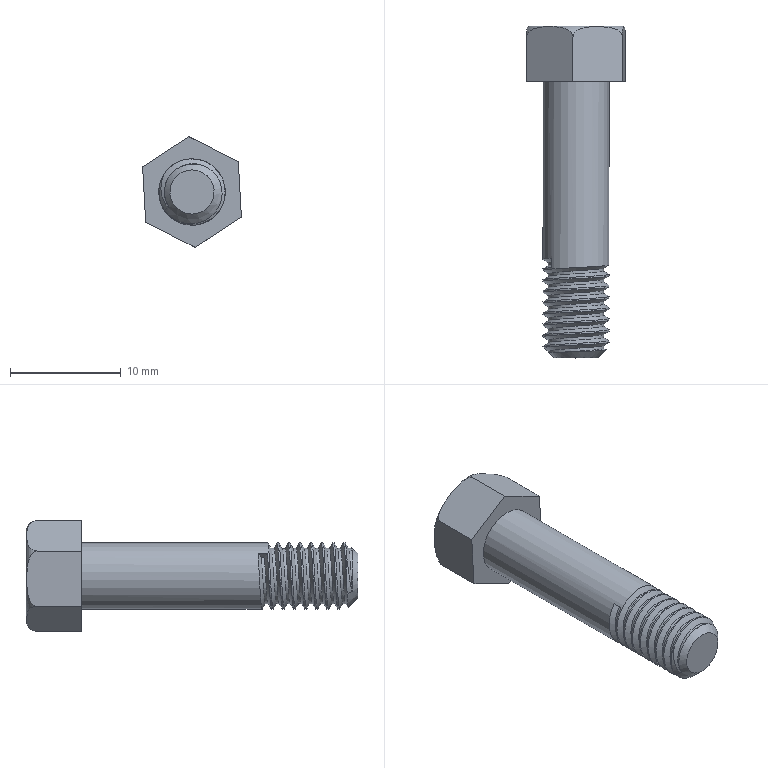Component | NX | JJZ-008_2 | 2 solids | 26 faces | volume 984 mm3 | plane 12 | cylinder 9 | cone 2 | spline 2 | torus 1 | commonest cylinder face diameters 6 x8 5 x1